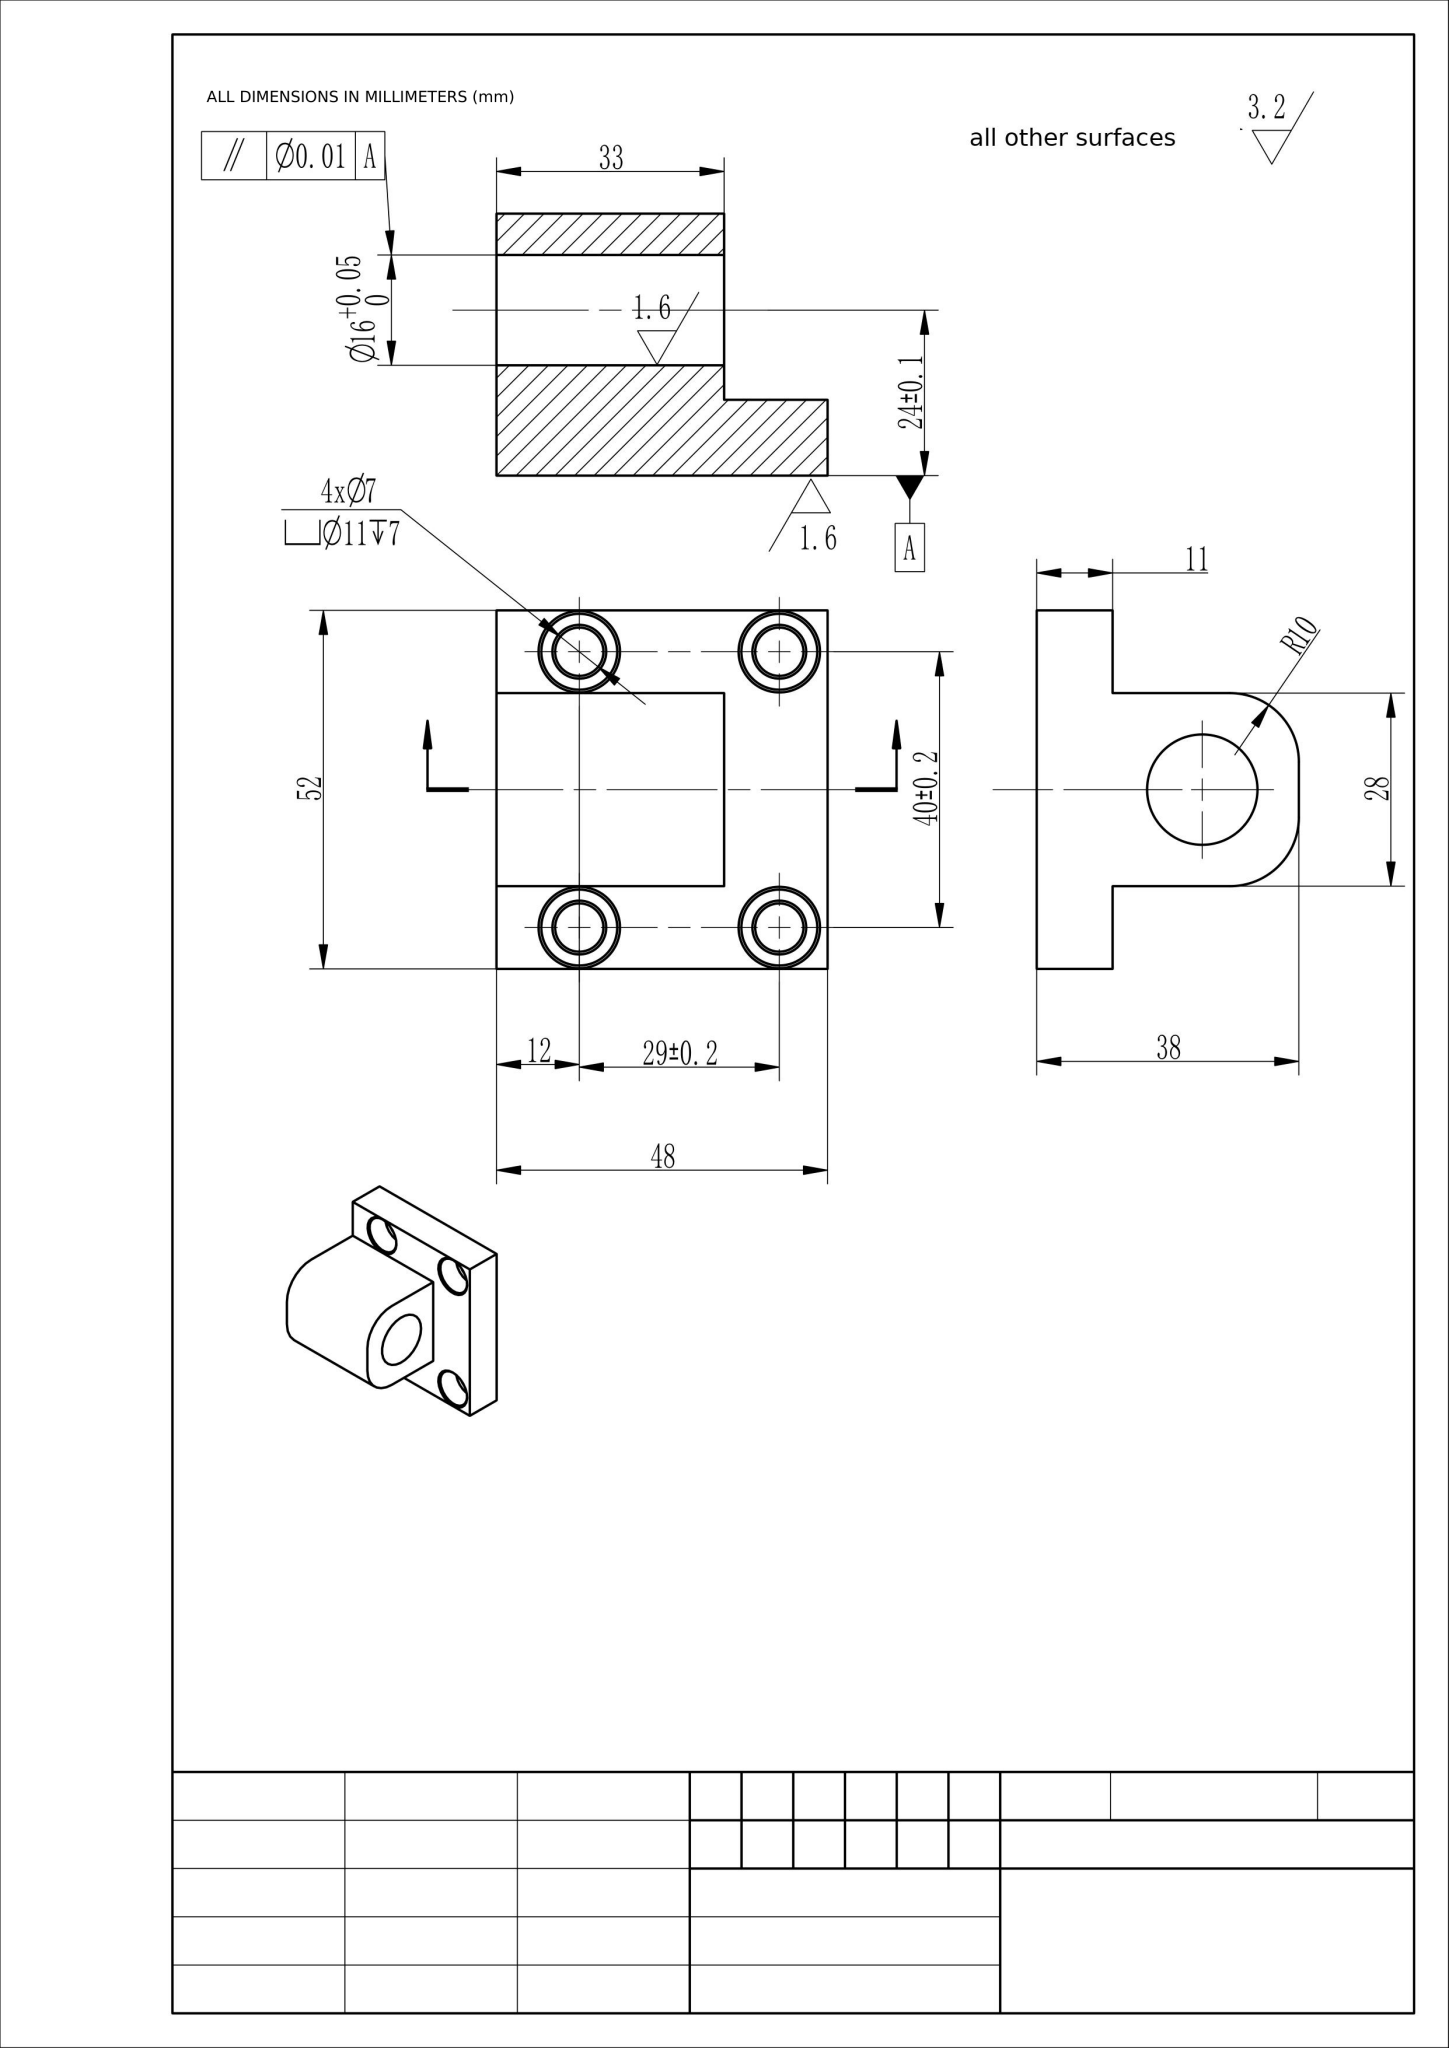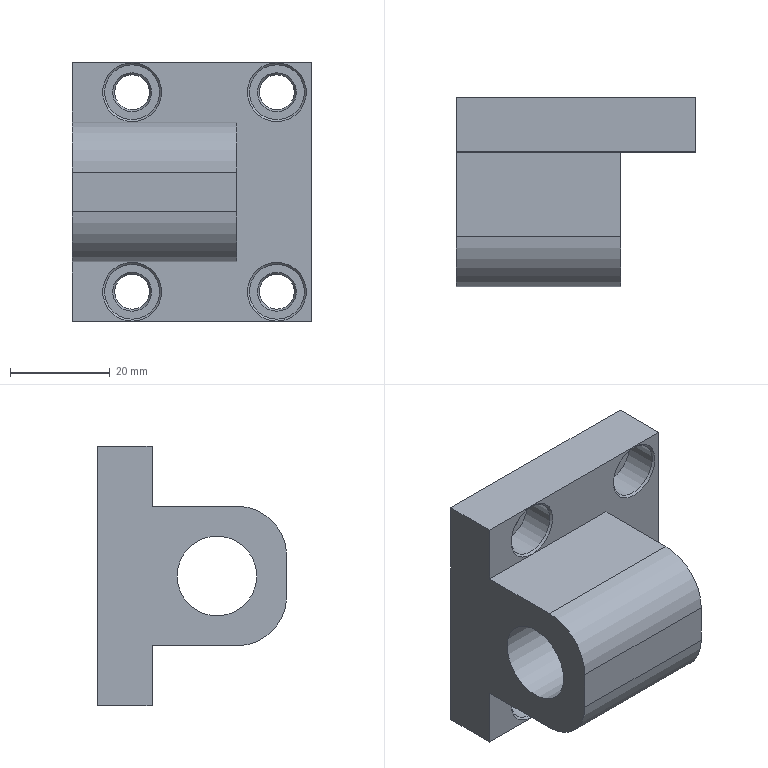Part | NX | mm | 1 solid | 37 faces | box 48 x 38 x 52 mm | volume 41090 mm3 | plane 14 | cone 12 | cylinder 11 | commonest cylinder face diameters 7 x4 11 x4 20 x2 16 x1
STEP:
#1=CARTESIAN_POINT('',(0.,0.,0.));
#2=DIRECTION('',(0.,0.,1.));
#3=DIRECTION('',(1.,0.,0.));
#4=AXIS2_PLACEMENT_3D('',#1,#2,#3);
#5=(LENGTH_UNIT()NAMED_UNIT(*)SI_UNIT(.MILLI.,.METRE.));
#6=UNCERTAINTY_MEASURE_WITH_UNIT(LENGTH_MEASURE(0.00002),#5,'','');
#7=(NAMED_UNIT(*)PLANE_ANGLE_UNIT()SI_UNIT($,.RADIAN.));
#8=PLANE_ANGLE_MEASURE_WITH_UNIT(PLANE_ANGLE_MEASURE(0.01745),#7);
#9=DIMENSIONAL_EXPONENTS(0.,0.,0.,0.,0.,0.,0.);
#10=(CONVERSION_BASED_UNIT('',#8)NAMED_UNIT(#9)PLANE_ANGLE_UNIT());
#11=(NAMED_UNIT(*)SI_UNIT($,.STERADIAN.)SOLID_ANGLE_UNIT());
#12=(GEOMETRIC_REPRESENTATION_CONTEXT(3)GLOBAL_UNCERTAINTY_ASSIGNED_CONTEXT((#6))GLOBAL_UNIT_ASSIGNED_CONTEXT((#5,#10,#11))REPRESENTATION_CONTEXT('',''));
#13=SHAPE_REPRESENTATION('',(#4),#12);
#14=CARTESIAN_POINT('',(0.,-14.,4.));
#15=VERTEX_POINT('',#14);
#16=CARTESIAN_POINT('',(0.,-14.,-4.));
#17=VERTEX_POINT('',#16);
#18=CARTESIAN_POINT('',(0.,-14.,14.));
#19=DIRECTION('',(0.,0.,-1.));
#20=VECTOR('',#19,1.);
#21=LINE('',#18,#20);
#22=EDGE_CURVE('',#15,#17,#21,.T.);
#23=ORIENTED_EDGE('',*,*,#22,.T.);
#24=CARTESIAN_POINT('',(33.,-14.,-4.));
#25=VERTEX_POINT('',#24);
#26=CARTESIAN_POINT('',(33.,-14.,-4.));
#27=DIRECTION('',(1.,0.,0.));
#28=VECTOR('',#27,1.);
#29=LINE('',#26,#28);
#30=EDGE_CURVE('',#17,#25,#29,.T.);
#31=ORIENTED_EDGE('',*,*,#30,.T.);
#32=CARTESIAN_POINT('',(33.,-14.,4.));
#33=VERTEX_POINT('',#32);
#34=CARTESIAN_POINT('',(33.,-14.,14.));
#35=DIRECTION('',(0.,0.,-1.));
#36=VECTOR('',#35,1.);
#37=LINE('',#34,#36);
#38=EDGE_CURVE('',#33,#25,#37,.T.);
#39=ORIENTED_EDGE('',*,*,#38,.F.);
#40=CARTESIAN_POINT('',(33.,-14.,4.));
#41=DIRECTION('',(-1.,0.,0.));
#42=VECTOR('',#41,1.);
#43=LINE('',#40,#42);
#44=EDGE_CURVE('',#33,#15,#43,.T.);
#45=ORIENTED_EDGE('',*,*,#44,.T.);
#46=EDGE_LOOP('',(#23,#31,#39,#45));
#47=FACE_OUTER_BOUND('',#46,.T.);
#48=CARTESIAN_POINT('',(33.,-14.,14.));
#49=DIRECTION('',(0.,1.,0.));
#50=DIRECTION('',(0.,0.,1.));
#51=AXIS2_PLACEMENT_3D('',#48,#49,#50);
#52=PLANE('',#51);
#53=ADVANCED_FACE('',(#47),#52,.F.);
#54=CARTESIAN_POINT('',(33.,-4.,-14.));
#55=VERTEX_POINT('',#54);
#56=CARTESIAN_POINT('',(33.,13.,-14.));
#57=VERTEX_POINT('',#56);
#58=CARTESIAN_POINT('',(33.,-14.,-14.));
#59=DIRECTION('',(0.,1.,0.));
#60=VECTOR('',#59,1.);
#61=LINE('',#58,#60);
#62=EDGE_CURVE('',#55,#57,#61,.T.);
#63=ORIENTED_EDGE('',*,*,#62,.F.);
#64=CARTESIAN_POINT('',(0.,-4.,-14.));
#65=VERTEX_POINT('',#64);
#66=CARTESIAN_POINT('',(33.,-4.,-14.));
#67=DIRECTION('',(-1.,0.,0.));
#68=VECTOR('',#67,1.);
#69=LINE('',#66,#68);
#70=EDGE_CURVE('',#55,#65,#69,.T.);
#71=ORIENTED_EDGE('',*,*,#70,.T.);
#72=CARTESIAN_POINT('',(0.,13.,-14.));
#73=VERTEX_POINT('',#72);
#74=CARTESIAN_POINT('',(0.,-14.,-14.));
#75=DIRECTION('',(0.,1.,0.));
#76=VECTOR('',#75,1.);
#77=LINE('',#74,#76);
#78=EDGE_CURVE('',#65,#73,#77,.T.);
#79=ORIENTED_EDGE('',*,*,#78,.T.);
#80=CARTESIAN_POINT('',(33.,13.,-14.));
#81=DIRECTION('',(-1.,0.,0.));
#82=VECTOR('',#81,1.);
#83=LINE('',#80,#82);
#84=EDGE_CURVE('',#57,#73,#83,.T.);
#85=ORIENTED_EDGE('',*,*,#84,.F.);
#86=EDGE_LOOP('',(#63,#71,#79,#85));
#87=FACE_OUTER_BOUND('',#86,.T.);
#88=CARTESIAN_POINT('',(33.,-14.,-14.));
#89=DIRECTION('',(0.,0.,1.));
#90=DIRECTION('',(1.,0.,0.));
#91=AXIS2_PLACEMENT_3D('',#88,#89,#90);
#92=PLANE('',#91);
#93=ADVANCED_FACE('',(#87),#92,.F.);
#94=CARTESIAN_POINT('',(0.,13.,-26.));
#95=VERTEX_POINT('',#94);
#96=CARTESIAN_POINT('',(0.,24.,-26.));
#97=VERTEX_POINT('',#96);
#98=CARTESIAN_POINT('',(0.,13.,-26.));
#99=DIRECTION('',(0.,1.,-0.));
#100=VECTOR('',#99,1.);
#101=LINE('',#98,#100);
#102=EDGE_CURVE('',#95,#97,#101,.T.);
#103=ORIENTED_EDGE('',*,*,#102,.T.);
#104=CARTESIAN_POINT('',(48.,24.,-26.));
#105=VERTEX_POINT('',#104);
#106=CARTESIAN_POINT('',(33.,24.,-26.));
#107=DIRECTION('',(-1.,0.,0.));
#108=VECTOR('',#107,1.);
#109=LINE('',#106,#108);
#110=EDGE_CURVE('',#105,#97,#109,.T.);
#111=ORIENTED_EDGE('',*,*,#110,.F.);
#112=CARTESIAN_POINT('',(48.,13.,-26.));
#113=VERTEX_POINT('',#112);
#114=CARTESIAN_POINT('',(48.,13.,-26.));
#115=DIRECTION('',(0.,1.,0.));
#116=VECTOR('',#115,1.);
#117=LINE('',#114,#116);
#118=EDGE_CURVE('',#113,#105,#117,.T.);
#119=ORIENTED_EDGE('',*,*,#118,.F.);
#120=CARTESIAN_POINT('',(33.,13.,-26.));
#121=DIRECTION('',(-1.,0.,0.));
#122=VECTOR('',#121,1.);
#123=LINE('',#120,#122);
#124=EDGE_CURVE('',#113,#95,#123,.T.);
#125=ORIENTED_EDGE('',*,*,#124,.T.);
#126=EDGE_LOOP('',(#103,#111,#119,#125));
#127=FACE_OUTER_BOUND('',#126,.T.);
#128=CARTESIAN_POINT('',(33.,13.,-26.));
#129=DIRECTION('',(0.,0.,1.));
#130=DIRECTION('',(0.,-1.,0.));
#131=AXIS2_PLACEMENT_3D('',#128,#129,#130);
#132=PLANE('',#131);
#133=ADVANCED_FACE('',(#127),#132,.F.);
#134=CARTESIAN_POINT('',(41.,24.,16.1));
#135=VERTEX_POINT('',#134);
#136=CARTESIAN_POINT('',(41.,24.,20.));
#137=DIRECTION('',(0.,-1.,0.));
#138=DIRECTION('',(0.,0.,-1.));
#139=AXIS2_PLACEMENT_3D('',#136,#137,#138);
#140=CIRCLE('',#139,3.9);
#141=EDGE_CURVE('',#135,#135,#140,.T.);
#142=ORIENTED_EDGE('',*,*,#141,.T.);
#143=EDGE_LOOP('',(#142));
#144=FACE_BOUND('',#143,.T.);
#145=CARTESIAN_POINT('',(41.,24.,-23.9));
#146=VERTEX_POINT('',#145);
#147=CARTESIAN_POINT('',(41.,24.,-20.));
#148=DIRECTION('',(0.,-1.,0.));
#149=DIRECTION('',(0.,0.,-1.));
#150=AXIS2_PLACEMENT_3D('',#147,#148,#149);
#151=CIRCLE('',#150,3.9);
#152=EDGE_CURVE('',#146,#146,#151,.T.);
#153=ORIENTED_EDGE('',*,*,#152,.T.);
#154=EDGE_LOOP('',(#153));
#155=FACE_BOUND('',#154,.T.);
#156=CARTESIAN_POINT('',(12.,24.,16.1));
#157=VERTEX_POINT('',#156);
#158=CARTESIAN_POINT('',(12.,24.,20.));
#159=DIRECTION('',(0.,-1.,0.));
#160=DIRECTION('',(0.,0.,-1.));
#161=AXIS2_PLACEMENT_3D('',#158,#159,#160);
#162=CIRCLE('',#161,3.9);
#163=EDGE_CURVE('',#157,#157,#162,.T.);
#164=ORIENTED_EDGE('',*,*,#163,.T.);
#165=EDGE_LOOP('',(#164));
#166=FACE_BOUND('',#165,.T.);
#167=CARTESIAN_POINT('',(12.,24.,-23.9));
#168=VERTEX_POINT('',#167);
#169=CARTESIAN_POINT('',(12.,24.,-20.));
#170=DIRECTION('',(0.,-1.,0.));
#171=DIRECTION('',(0.,0.,-1.));
#172=AXIS2_PLACEMENT_3D('',#169,#170,#171);
#173=CIRCLE('',#172,3.9);
#174=EDGE_CURVE('',#168,#168,#173,.T.);
#175=ORIENTED_EDGE('',*,*,#174,.T.);
#176=EDGE_LOOP('',(#175));
#177=FACE_BOUND('',#176,.T.);
#178=CARTESIAN_POINT('',(0.,24.,26.));
#179=VERTEX_POINT('',#178);
#180=CARTESIAN_POINT('',(0.,24.,-26.));
#181=DIRECTION('',(0.,0.,1.));
#182=VECTOR('',#181,1.);
#183=LINE('',#180,#182);
#184=EDGE_CURVE('',#97,#179,#183,.T.);
#185=ORIENTED_EDGE('',*,*,#184,.T.);
#186=CARTESIAN_POINT('',(48.,24.,26.));
#187=VERTEX_POINT('',#186);
#188=CARTESIAN_POINT('',(33.,24.,26.));
#189=DIRECTION('',(-1.,0.,0.));
#190=VECTOR('',#189,1.);
#191=LINE('',#188,#190);
#192=EDGE_CURVE('',#187,#179,#191,.T.);
#193=ORIENTED_EDGE('',*,*,#192,.F.);
#194=CARTESIAN_POINT('',(48.,24.,-26.));
#195=DIRECTION('',(0.,0.,1.));
#196=VECTOR('',#195,1.);
#197=LINE('',#194,#196);
#198=EDGE_CURVE('',#105,#187,#197,.T.);
#199=ORIENTED_EDGE('',*,*,#198,.F.);
#200=ORIENTED_EDGE('',*,*,#110,.T.);
#201=EDGE_LOOP('',(#185,#193,#199,#200));
#202=FACE_BOUND('',#201,.T.);
#203=CARTESIAN_POINT('',(33.,24.,-26.));
#204=DIRECTION('',(0.,-1.,0.));
#205=DIRECTION('',(0.,0.,-1.));
#206=AXIS2_PLACEMENT_3D('',#203,#204,#205);
#207=PLANE('',#206);
#208=ADVANCED_FACE('',(#144,#155,#166,#177,#202),#207,.F.);
#209=CARTESIAN_POINT('',(0.,13.,26.));
#210=VERTEX_POINT('',#209);
#211=CARTESIAN_POINT('',(0.,24.,26.));
#212=DIRECTION('',(0.,-1.,0.));
#213=VECTOR('',#212,1.);
#214=LINE('',#211,#213);
#215=EDGE_CURVE('',#179,#210,#214,.T.);
#216=ORIENTED_EDGE('',*,*,#215,.T.);
#217=CARTESIAN_POINT('',(48.,13.,26.));
#218=VERTEX_POINT('',#217);
#219=CARTESIAN_POINT('',(33.,13.,26.));
#220=DIRECTION('',(-1.,0.,0.));
#221=VECTOR('',#220,1.);
#222=LINE('',#219,#221);
#223=EDGE_CURVE('',#218,#210,#222,.T.);
#224=ORIENTED_EDGE('',*,*,#223,.F.);
#225=CARTESIAN_POINT('',(48.,24.,26.));
#226=DIRECTION('',(0.,-1.,-0.));
#227=VECTOR('',#226,1.);
#228=LINE('',#225,#227);
#229=EDGE_CURVE('',#187,#218,#228,.T.);
#230=ORIENTED_EDGE('',*,*,#229,.F.);
#231=ORIENTED_EDGE('',*,*,#192,.T.);
#232=EDGE_LOOP('',(#216,#224,#230,#231));
#233=FACE_OUTER_BOUND('',#232,.T.);
#234=CARTESIAN_POINT('',(33.,24.,26.));
#235=DIRECTION('',(0.,0.,-1.));
#236=DIRECTION('',(-1.,0.,0.));
#237=AXIS2_PLACEMENT_3D('',#234,#235,#236);
#238=PLANE('',#237);
#239=ADVANCED_FACE('',(#233),#238,.F.);
#240=CARTESIAN_POINT('',(41.,13.,25.9));
#241=VERTEX_POINT('',#240);
#242=CARTESIAN_POINT('',(41.,13.,20.));
#243=DIRECTION('',(0.,1.,0.));
#244=DIRECTION('',(0.,0.,1.));
#245=AXIS2_PLACEMENT_3D('',#242,#243,#244);
#246=CIRCLE('',#245,5.9);
#247=EDGE_CURVE('',#241,#241,#246,.T.);
#248=ORIENTED_EDGE('',*,*,#247,.T.);
#249=EDGE_LOOP('',(#248));
#250=FACE_BOUND('',#249,.T.);
#251=CARTESIAN_POINT('',(41.,13.,-14.1));
#252=VERTEX_POINT('',#251);
#253=CARTESIAN_POINT('',(41.,13.,-20.));
#254=DIRECTION('',(0.,1.,0.));
#255=DIRECTION('',(0.,0.,1.));
#256=AXIS2_PLACEMENT_3D('',#253,#254,#255);
#257=CIRCLE('',#256,5.9);
#258=EDGE_CURVE('',#252,#252,#257,.T.);
#259=ORIENTED_EDGE('',*,*,#258,.T.);
#260=EDGE_LOOP('',(#259));
#261=FACE_BOUND('',#260,.T.);
#262=CARTESIAN_POINT('',(12.,13.,25.9));
#263=VERTEX_POINT('',#262);
#264=CARTESIAN_POINT('',(12.,13.,20.));
#265=DIRECTION('',(0.,1.,0.));
#266=DIRECTION('',(0.,0.,1.));
#267=AXIS2_PLACEMENT_3D('',#264,#265,#266);
#268=CIRCLE('',#267,5.9);
#269=EDGE_CURVE('',#263,#263,#268,.T.);
#270=ORIENTED_EDGE('',*,*,#269,.T.);
#271=EDGE_LOOP('',(#270));
#272=FACE_BOUND('',#271,.T.);
#273=CARTESIAN_POINT('',(12.,13.,-14.1));
#274=VERTEX_POINT('',#273);
#275=CARTESIAN_POINT('',(12.,13.,-20.));
#276=DIRECTION('',(0.,1.,0.));
#277=DIRECTION('',(0.,0.,1.));
#278=AXIS2_PLACEMENT_3D('',#275,#276,#277);
#279=CIRCLE('',#278,5.9);
#280=EDGE_CURVE('',#274,#274,#279,.T.);
#281=ORIENTED_EDGE('',*,*,#280,.T.);
#282=EDGE_LOOP('',(#281));
#283=FACE_BOUND('',#282,.T.);
#284=CARTESIAN_POINT('',(0.,13.,14.));
#285=VERTEX_POINT('',#284);
#286=CARTESIAN_POINT('',(0.,13.,26.));
#287=DIRECTION('',(0.,0.,-1.));
#288=VECTOR('',#287,1.);
#289=LINE('',#286,#288);
#290=EDGE_CURVE('',#210,#285,#289,.T.);
#291=ORIENTED_EDGE('',*,*,#290,.T.);
#292=CARTESIAN_POINT('',(33.,13.,14.));
#293=VERTEX_POINT('',#292);
#294=CARTESIAN_POINT('',(33.,13.,14.));
#295=DIRECTION('',(-1.,0.,0.));
#296=VECTOR('',#295,1.);
#297=LINE('',#294,#296);
#298=EDGE_CURVE('',#293,#285,#297,.T.);
#299=ORIENTED_EDGE('',*,*,#298,.F.);
#300=CARTESIAN_POINT('',(33.,13.,26.));
#301=DIRECTION('',(0.,0.,1.));
#302=VECTOR('',#301,1.);
#303=LINE('',#300,#302);
#304=EDGE_CURVE('',#57,#293,#303,.T.);
#305=ORIENTED_EDGE('',*,*,#304,.F.);
#306=ORIENTED_EDGE('',*,*,#84,.T.);
#307=CARTESIAN_POINT('',(0.,13.,-14.));
#308=DIRECTION('',(0.,0.,-1.));
#309=VECTOR('',#308,1.);
#310=LINE('',#307,#309);
#311=EDGE_CURVE('',#73,#95,#310,.T.);
#312=ORIENTED_EDGE('',*,*,#311,.T.);
#313=ORIENTED_EDGE('',*,*,#124,.F.);
#314=CARTESIAN_POINT('',(48.,13.,26.));
#315=DIRECTION('',(0.,-0.,-1.));
#316=VECTOR('',#315,1.);
#317=LINE('',#314,#316);
#318=EDGE_CURVE('',#218,#113,#317,.T.);
#319=ORIENTED_EDGE('',*,*,#318,.F.);
#320=ORIENTED_EDGE('',*,*,#223,.T.);
#321=EDGE_LOOP('',(#291,#299,#305,#306,#312,#313,#319,#320));
#322=FACE_BOUND('',#321,.T.);
#323=CARTESIAN_POINT('',(33.,13.,26.));
#324=DIRECTION('',(0.,1.,0.));
#325=DIRECTION('',(0.,0.,1.));
#326=AXIS2_PLACEMENT_3D('',#323,#324,#325);
#327=PLANE('',#326);
#328=ADVANCED_FACE('',(#250,#261,#272,#283,#322),#327,.F.);
#329=CARTESIAN_POINT('',(0.,-4.,14.));
#330=VERTEX_POINT('',#329);
#331=CARTESIAN_POINT('',(0.,13.,14.));
#332=DIRECTION('',(0.,-1.,0.));
#333=VECTOR('',#332,1.);
#334=LINE('',#331,#333);
#335=EDGE_CURVE('',#285,#330,#334,.T.);
#336=ORIENTED_EDGE('',*,*,#335,.T.);
#337=CARTESIAN_POINT('',(33.,-4.,14.));
#338=VERTEX_POINT('',#337);
#339=CARTESIAN_POINT('',(33.,-4.,14.));
#340=DIRECTION('',(1.,0.,0.));
#341=VECTOR('',#340,1.);
#342=LINE('',#339,#341);
#343=EDGE_CURVE('',#330,#338,#342,.T.);
#344=ORIENTED_EDGE('',*,*,#343,.T.);
#345=CARTESIAN_POINT('',(33.,13.,14.));
#346=DIRECTION('',(0.,-1.,0.));
#347=VECTOR('',#346,1.);
#348=LINE('',#345,#347);
#349=EDGE_CURVE('',#293,#338,#348,.T.);
#350=ORIENTED_EDGE('',*,*,#349,.F.);
#351=ORIENTED_EDGE('',*,*,#298,.T.);
#352=EDGE_LOOP('',(#336,#344,#350,#351));
#353=FACE_OUTER_BOUND('',#352,.T.);
#354=CARTESIAN_POINT('',(33.,13.,14.));
#355=DIRECTION('',(0.,0.,-1.));
#356=DIRECTION('',(-1.,0.,0.));
#357=AXIS2_PLACEMENT_3D('',#354,#355,#356);
#358=PLANE('',#357);
#359=ADVANCED_FACE('',(#353),#358,.F.);
#360=CARTESIAN_POINT('',(33.,8.,-0.));
#361=VERTEX_POINT('',#360);
#362=CARTESIAN_POINT('',(33.,0.,0.));
#363=DIRECTION('',(1.,0.,0.));
#364=DIRECTION('',(0.,1.,-0.));
#365=AXIS2_PLACEMENT_3D('',#362,#363,#364);
#366=CIRCLE('',#365,8.);
#367=EDGE_CURVE('',#361,#361,#366,.T.);
#368=ORIENTED_EDGE('',*,*,#367,.T.);
#369=EDGE_LOOP('',(#368));
#370=FACE_BOUND('',#369,.T.);
#371=CARTESIAN_POINT('',(0.,8.,-0.));
#372=VERTEX_POINT('',#371);
#373=CARTESIAN_POINT('',(0.,0.,0.));
#374=DIRECTION('',(1.,0.,0.));
#375=DIRECTION('',(0.,1.,-0.));
#376=AXIS2_PLACEMENT_3D('',#373,#374,#375);
#377=CIRCLE('',#376,8.);
#378=EDGE_CURVE('',#372,#372,#377,.T.);
#379=ORIENTED_EDGE('',*,*,#378,.F.);
#380=EDGE_LOOP('',(#379));
#381=FACE_BOUND('',#380,.T.);
#382=CARTESIAN_POINT('',(33.,0.,0.));
#383=DIRECTION('',(-1.,0.,0.));
#384=DIRECTION('',(0.,0.,1.));
#385=AXIS2_PLACEMENT_3D('',#382,#383,#384);
#386=CYLINDRICAL_SURFACE('',#385,8.);
#387=ADVANCED_FACE('',(#370,#381),#386,.F.);
#388=ORIENTED_EDGE('',*,*,#304,.T.);
#389=ORIENTED_EDGE('',*,*,#349,.T.);
#390=CARTESIAN_POINT('',(33.,-4.,4.));
#391=DIRECTION('',(1.,0.,0.));
#392=DIRECTION('',(0.,0.,-1.));
#393=AXIS2_PLACEMENT_3D('',#390,#391,#392);
#394=CIRCLE('',#393,10.);
#395=EDGE_CURVE('',#338,#33,#394,.T.);
#396=ORIENTED_EDGE('',*,*,#395,.T.);
#397=ORIENTED_EDGE('',*,*,#38,.T.);
#398=CARTESIAN_POINT('',(33.,-4.,-4.));
#399=DIRECTION('',(1.,0.,0.));
#400=DIRECTION('',(0.,0.,-1.));
#401=AXIS2_PLACEMENT_3D('',#398,#399,#400);
#402=CIRCLE('',#401,10.);
#403=EDGE_CURVE('',#25,#55,#402,.T.);
#404=ORIENTED_EDGE('',*,*,#403,.T.);
#405=ORIENTED_EDGE('',*,*,#62,.T.);
#406=EDGE_LOOP('',(#388,#389,#396,#397,#404,#405));
#407=FACE_BOUND('',#406,.T.);
#408=ORIENTED_EDGE('',*,*,#367,.F.);
#409=EDGE_LOOP('',(#408));
#410=FACE_BOUND('',#409,.T.);
#411=CARTESIAN_POINT('',(33.,0.,0.));
#412=DIRECTION('',(1.,0.,0.));
#413=DIRECTION('',(0.,0.,-1.));
#414=AXIS2_PLACEMENT_3D('',#411,#412,#413);
#415=PLANE('',#414);
#416=ADVANCED_FACE('',(#407,#410),#415,.T.);
#417=ORIENTED_EDGE('',*,*,#78,.F.);
#418=CARTESIAN_POINT('',(0.,-4.,-4.));
#419=DIRECTION('',(-1.,0.,0.));
#420=DIRECTION('',(0.,0.,-1.));
#421=AXIS2_PLACEMENT_3D('',#418,#419,#420);
#422=CIRCLE('',#421,10.);
#423=EDGE_CURVE('',#65,#17,#422,.T.);
#424=ORIENTED_EDGE('',*,*,#423,.T.);
#425=ORIENTED_EDGE('',*,*,#22,.F.);
#426=CARTESIAN_POINT('',(0.,-4.,4.));
#427=DIRECTION('',(-1.,0.,0.));
#428=DIRECTION('',(0.,0.,-1.));
#429=AXIS2_PLACEMENT_3D('',#426,#427,#428);
#430=CIRCLE('',#429,10.);
#431=EDGE_CURVE('',#15,#330,#430,.T.);
#432=ORIENTED_EDGE('',*,*,#431,.T.);
#433=ORIENTED_EDGE('',*,*,#335,.F.);
#434=ORIENTED_EDGE('',*,*,#290,.F.);
#435=ORIENTED_EDGE('',*,*,#215,.F.);
#436=ORIENTED_EDGE('',*,*,#184,.F.);
#437=ORIENTED_EDGE('',*,*,#102,.F.);
#438=ORIENTED_EDGE('',*,*,#311,.F.);
#439=EDGE_LOOP('',(#417,#424,#425,#432,#433,#434,#435,#436,#437,#438));
#440=FACE_BOUND('',#439,.T.);
#441=ORIENTED_EDGE('',*,*,#378,.T.);
#442=EDGE_LOOP('',(#441));
#443=FACE_BOUND('',#442,.T.);
#444=CARTESIAN_POINT('',(0.,0.,0.));
#445=DIRECTION('',(1.,0.,0.));
#446=DIRECTION('',(0.,0.,-1.));
#447=AXIS2_PLACEMENT_3D('',#444,#445,#446);
#448=PLANE('',#447);
#449=ADVANCED_FACE('',(#440,#443),#448,.F.);
#450=ORIENTED_EDGE('',*,*,#403,.F.);
#451=ORIENTED_EDGE('',*,*,#30,.F.);
#452=ORIENTED_EDGE('',*,*,#423,.F.);
#453=ORIENTED_EDGE('',*,*,#70,.F.);
#454=EDGE_LOOP('',(#450,#451,#452,#453));
#455=FACE_OUTER_BOUND('',#454,.T.);
#456=CARTESIAN_POINT('',(33.,-4.,-4.));
#457=DIRECTION('',(-1.,0.,0.));
#458=DIRECTION('',(0.,0.,1.));
#459=AXIS2_PLACEMENT_3D('',#456,#457,#458);
#460=CYLINDRICAL_SURFACE('',#459,10.);
#461=ADVANCED_FACE('',(#455),#460,.T.);
#462=ORIENTED_EDGE('',*,*,#395,.F.);
#463=ORIENTED_EDGE('',*,*,#343,.F.);
#464=ORIENTED_EDGE('',*,*,#431,.F.);
#465=ORIENTED_EDGE('',*,*,#44,.F.);
#466=EDGE_LOOP('',(#462,#463,#464,#465));
#467=FACE_OUTER_BOUND('',#466,.T.);
#468=CARTESIAN_POINT('',(33.,-4.,4.));
#469=DIRECTION('',(-1.,0.,0.));
#470=DIRECTION('',(0.,0.,1.));
#471=AXIS2_PLACEMENT_3D('',#468,#469,#470);
#472=CYLINDRICAL_SURFACE('',#471,10.);
#473=ADVANCED_FACE('',(#467),#472,.T.);
#474=ORIENTED_EDGE('',*,*,#318,.T.);
#475=ORIENTED_EDGE('',*,*,#118,.T.);
#476=ORIENTED_EDGE('',*,*,#198,.T.);
#477=ORIENTED_EDGE('',*,*,#229,.T.);
#478=EDGE_LOOP('',(#474,#475,#476,#477));
#479=FACE_OUTER_BOUND('',#478,.T.);
#480=CARTESIAN_POINT('',(48.,0.,0.));
#481=DIRECTION('',(1.,0.,0.));
#482=DIRECTION('',(0.,0.,-1.));
#483=AXIS2_PLACEMENT_3D('',#480,#481,#482);
#484=PLANE('',#483);
#485=ADVANCED_FACE('',(#479),#484,.T.);
#486=CARTESIAN_POINT('',(12.,23.6,-23.5));
#487=VERTEX_POINT('',#486);
#488=CARTESIAN_POINT('',(12.,23.6,-20.));
#489=DIRECTION('',(0.,1.,0.));
#490=DIRECTION('',(0.,0.,-1.));
#491=AXIS2_PLACEMENT_3D('',#488,#489,#490);
#492=CIRCLE('',#491,3.5);
#493=EDGE_CURVE('',#487,#487,#492,.T.);
#494=ORIENTED_EDGE('',*,*,#493,.T.);
#495=EDGE_LOOP('',(#494));
#496=FACE_BOUND('',#495,.T.);
#497=CARTESIAN_POINT('',(12.,20.493,-16.5));
#498=VERTEX_POINT('',#497);
#499=CARTESIAN_POINT('',(12.,20.493,-20.));
#500=DIRECTION('',(0.,-1.,0.));
#501=DIRECTION('',(0.,0.,1.));
#502=AXIS2_PLACEMENT_3D('',#499,#500,#501);
#503=CIRCLE('',#502,3.5);
#504=EDGE_CURVE('',#498,#498,#503,.T.);
#505=ORIENTED_EDGE('',*,*,#504,.T.);
#506=EDGE_LOOP('',(#505));
#507=FACE_BOUND('',#506,.T.);
#508=CARTESIAN_POINT('',(12.,93.,-20.));
#509=DIRECTION('',(0.,1.,0.));
#510=DIRECTION('',(0.,0.,1.));
#511=AXIS2_PLACEMENT_3D('',#508,#509,#510);
#512=CYLINDRICAL_SURFACE('',#511,3.5);
#513=ADVANCED_FACE('',(#496,#507),#512,.F.);
#514=CARTESIAN_POINT('',(12.,19.8,-16.1));
#515=VERTEX_POINT('',#514);
#516=CARTESIAN_POINT('',(12.,19.8,-20.));
#517=DIRECTION('',(0.,1.,0.));
#518=DIRECTION('',(0.,0.,1.));
#519=AXIS2_PLACEMENT_3D('',#516,#517,#518);
#520=CIRCLE('',#519,3.9);
#521=EDGE_CURVE('',#515,#515,#520,.T.);
#522=ORIENTED_EDGE('',*,*,#521,.T.);
#523=EDGE_LOOP('',(#522));
#524=FACE_BOUND('',#523,.T.);
#525=CARTESIAN_POINT('',(12.,19.8,-14.5));
#526=VERTEX_POINT('',#525);
#527=CARTESIAN_POINT('',(12.,19.8,-20.));
#528=DIRECTION('',(0.,-1.,-0.));
#529=DIRECTION('',(0.,0.,1.));
#530=AXIS2_PLACEMENT_3D('',#527,#528,#529);
#531=CIRCLE('',#530,5.5);
#532=EDGE_CURVE('',#526,#526,#531,.T.);
#533=ORIENTED_EDGE('',*,*,#532,.T.);
#534=EDGE_LOOP('',(#533));
#535=FACE_BOUND('',#534,.T.);
#536=CARTESIAN_POINT('',(12.,19.8,-20.));
#537=DIRECTION('',(0.,1.,0.));
#538=DIRECTION('',(0.,-0.,1.));
#539=AXIS2_PLACEMENT_3D('',#536,#537,#538);
#540=PLANE('',#539);
#541=ADVANCED_FACE('',(#524,#535),#540,.F.);
#542=CARTESIAN_POINT('',(12.,13.4,-14.5));
#543=VERTEX_POINT('',#542);
#544=CARTESIAN_POINT('',(12.,13.4,-20.));
#545=DIRECTION('',(0.,-1.,0.));
#546=DIRECTION('',(0.,0.,1.));
#547=AXIS2_PLACEMENT_3D('',#544,#545,#546);
#548=CIRCLE('',#547,5.5);
#549=EDGE_CURVE('',#543,#543,#548,.T.);
#550=ORIENTED_EDGE('',*,*,#549,.T.);
#551=EDGE_LOOP('',(#550));
#552=FACE_BOUND('',#551,.T.);
#553=ORIENTED_EDGE('',*,*,#532,.F.);
#554=EDGE_LOOP('',(#553));
#555=FACE_BOUND('',#554,.T.);
#556=CARTESIAN_POINT('',(12.,13.,-20.));
#557=DIRECTION('',(0.,1.,0.));
#558=DIRECTION('',(0.,0.,1.));
#559=AXIS2_PLACEMENT_3D('',#556,#557,#558);
#560=CYLINDRICAL_SURFACE('',#559,5.5);
#561=ADVANCED_FACE('',(#552,#555),#560,.F.);
#562=ORIENTED_EDGE('',*,*,#521,.F.);
#563=EDGE_LOOP('',(#562));
#564=FACE_BOUND('',#563,.T.);
#565=ORIENTED_EDGE('',*,*,#504,.F.);
#566=EDGE_LOOP('',(#565));
#567=FACE_BOUND('',#566,.T.);
#568=CARTESIAN_POINT('',(12.,20.493,-20.));
#569=DIRECTION('',(0.,-1.,0.));
#570=DIRECTION('',(0.,0.,-1.));
#571=AXIS2_PLACEMENT_3D('',#568,#569,#570);
#572=CONICAL_SURFACE('',#571,3.5,30.);
#573=ADVANCED_FACE('',(#564,#567),#572,.F.);
#574=ORIENTED_EDGE('',*,*,#549,.F.);
#575=EDGE_LOOP('',(#574));
#576=FACE_BOUND('',#575,.T.);
#577=ORIENTED_EDGE('',*,*,#280,.F.);
#578=EDGE_LOOP('',(#577));
#579=FACE_BOUND('',#578,.T.);
#580=CARTESIAN_POINT('',(12.,13.,-20.));
#581=DIRECTION('',(0.,-1.,0.));
#582=DIRECTION('',(0.,0.,-1.));
#583=AXIS2_PLACEMENT_3D('',#580,#581,#582);
#584=CONICAL_SURFACE('',#583,5.9,45.);
#585=ADVANCED_FACE('',(#576,#579),#584,.F.);
#586=ORIENTED_EDGE('',*,*,#493,.F.);
#587=EDGE_LOOP('',(#586));
#588=FACE_BOUND('',#587,.T.);
#589=ORIENTED_EDGE('',*,*,#174,.F.);
#590=EDGE_LOOP('',(#589));
#591=FACE_BOUND('',#590,.T.);
#592=CARTESIAN_POINT('',(12.,24.,-20.));
#593=DIRECTION('',(0.,1.,0.));
#594=DIRECTION('',(0.,0.,1.));
#595=AXIS2_PLACEMENT_3D('',#592,#593,#594);
#596=CONICAL_SURFACE('',#595,3.9,45.);
#597=ADVANCED_FACE('',(#588,#591),#596,.F.);
#598=CARTESIAN_POINT('',(12.,23.6,16.5));
#599=VERTEX_POINT('',#598);
#600=CARTESIAN_POINT('',(12.,23.6,20.));
#601=DIRECTION('',(0.,1.,0.));
#602=DIRECTION('',(0.,0.,-1.));
#603=AXIS2_PLACEMENT_3D('',#600,#601,#602);
#604=CIRCLE('',#603,3.5);
#605=EDGE_CURVE('',#599,#599,#604,.T.);
#606=ORIENTED_EDGE('',*,*,#605,.T.);
#607=EDGE_LOOP('',(#606));
#608=FACE_BOUND('',#607,.T.);
#609=CARTESIAN_POINT('',(12.,20.493,23.5));
#610=VERTEX_POINT('',#609);
#611=CARTESIAN_POINT('',(12.,20.493,20.));
#612=DIRECTION('',(0.,-1.,0.));
#613=DIRECTION('',(0.,0.,1.));
#614=AXIS2_PLACEMENT_3D('',#611,#612,#613);
#615=CIRCLE('',#614,3.5);
#616=EDGE_CURVE('',#610,#610,#615,.T.);
#617=ORIENTED_EDGE('',*,*,#616,.T.);
#618=EDGE_LOOP('',(#617));
#619=FACE_BOUND('',#618,.T.);
#620=CARTESIAN_POINT('',(12.,93.,20.));
#621=DIRECTION('',(0.,1.,0.));
#622=DIRECTION('',(0.,0.,1.));
#623=AXIS2_PLACEMENT_3D('',#620,#621,#622);
#624=CYLINDRICAL_SURFACE('',#623,3.5);
#625=ADVANCED_FACE('',(#608,#619),#624,.F.);
#626=CARTESIAN_POINT('',(12.,19.8,23.9));
#627=VERTEX_POINT('',#626);
#628=CARTESIAN_POINT('',(12.,19.8,20.));
#629=DIRECTION('',(0.,1.,0.));
#630=DIRECTION('',(0.,0.,1.));
#631=AXIS2_PLACEMENT_3D('',#628,#629,#630);
#632=CIRCLE('',#631,3.9);
#633=EDGE_CURVE('',#627,#627,#632,.T.);
#634=ORIENTED_EDGE('',*,*,#633,.T.);
#635=EDGE_LOOP('',(#634));
#636=FACE_BOUND('',#635,.T.);
#637=CARTESIAN_POINT('',(12.,19.8,25.5));
#638=VERTEX_POINT('',#637);
#639=CARTESIAN_POINT('',(12.,19.8,20.));
#640=DIRECTION('',(0.,-1.,-0.));
#641=DIRECTION('',(0.,0.,1.));
#642=AXIS2_PLACEMENT_3D('',#639,#640,#641);
#643=CIRCLE('',#642,5.5);
#644=EDGE_CURVE('',#638,#638,#643,.T.);
#645=ORIENTED_EDGE('',*,*,#644,.T.);
#646=EDGE_LOOP('',(#645));
#647=FACE_BOUND('',#646,.T.);
#648=CARTESIAN_POINT('',(12.,19.8,20.));
#649=DIRECTION('',(0.,1.,0.));
#650=DIRECTION('',(0.,-0.,1.));
#651=AXIS2_PLACEMENT_3D('',#648,#649,#650);
#652=PLANE('',#651);
#653=ADVANCED_FACE('',(#636,#647),#652,.F.);
#654=CARTESIAN_POINT('',(12.,13.4,25.5));
#655=VERTEX_POINT('',#654);
#656=CARTESIAN_POINT('',(12.,13.4,20.));
#657=DIRECTION('',(0.,-1.,0.));
#658=DIRECTION('',(0.,0.,1.));
#659=AXIS2_PLACEMENT_3D('',#656,#657,#658);
#660=CIRCLE('',#659,5.5);
#661=EDGE_CURVE('',#655,#655,#660,.T.);
#662=ORIENTED_EDGE('',*,*,#661,.T.);
#663=EDGE_LOOP('',(#662));
#664=FACE_BOUND('',#663,.T.);
#665=ORIENTED_EDGE('',*,*,#644,.F.);
#666=EDGE_LOOP('',(#665));
#667=FACE_BOUND('',#666,.T.);
#668=CARTESIAN_POINT('',(12.,13.,20.));
#669=DIRECTION('',(0.,1.,0.));
#670=DIRECTION('',(0.,0.,1.));
#671=AXIS2_PLACEMENT_3D('',#668,#669,#670);
#672=CYLINDRICAL_SURFACE('',#671,5.5);
#673=ADVANCED_FACE('',(#664,#667),#672,.F.);
#674=ORIENTED_EDGE('',*,*,#633,.F.);
#675=EDGE_LOOP('',(#674));
#676=FACE_BOUND('',#675,.T.);
#677=ORIENTED_EDGE('',*,*,#616,.F.);
#678=EDGE_LOOP('',(#677));
#679=FACE_BOUND('',#678,.T.);
#680=CARTESIAN_POINT('',(12.,20.493,20.));
#681=DIRECTION('',(0.,-1.,0.));
#682=DIRECTION('',(0.,0.,-1.));
#683=AXIS2_PLACEMENT_3D('',#680,#681,#682);
#684=CONICAL_SURFACE('',#683,3.5,30.);
#685=ADVANCED_FACE('',(#676,#679),#684,.F.);
#686=ORIENTED_EDGE('',*,*,#661,.F.);
#687=EDGE_LOOP('',(#686));
#688=FACE_BOUND('',#687,.T.);
#689=ORIENTED_EDGE('',*,*,#269,.F.);
#690=EDGE_LOOP('',(#689));
#691=FACE_BOUND('',#690,.T.);
#692=CARTESIAN_POINT('',(12.,13.,20.));
#693=DIRECTION('',(0.,-1.,0.));
#694=DIRECTION('',(0.,0.,-1.));
#695=AXIS2_PLACEMENT_3D('',#692,#693,#694);
#696=CONICAL_SURFACE('',#695,5.9,45.);
#697=ADVANCED_FACE('',(#688,#691),#696,.F.);
#698=ORIENTED_EDGE('',*,*,#605,.F.);
#699=EDGE_LOOP('',(#698));
#700=FACE_BOUND('',#699,.T.);
#701=ORIENTED_EDGE('',*,*,#163,.F.);
#702=EDGE_LOOP('',(#701));
#703=FACE_BOUND('',#702,.T.);
#704=CARTESIAN_POINT('',(12.,24.,20.));
#705=DIRECTION('',(0.,1.,0.));
#706=DIRECTION('',(0.,0.,1.));
#707=AXIS2_PLACEMENT_3D('',#704,#705,#706);
#708=CONICAL_SURFACE('',#707,3.9,45.);
#709=ADVANCED_FACE('',(#700,#703),#708,.F.);
#710=CARTESIAN_POINT('',(41.,23.6,-23.5));
#711=VERTEX_POINT('',#710);
#712=CARTESIAN_POINT('',(41.,23.6,-20.));
#713=DIRECTION('',(0.,1.,0.));
#714=DIRECTION('',(0.,0.,-1.));
#715=AXIS2_PLACEMENT_3D('',#712,#713,#714);
#716=CIRCLE('',#715,3.5);
#717=EDGE_CURVE('',#711,#711,#716,.T.);
#718=ORIENTED_EDGE('',*,*,#717,.T.);
#719=EDGE_LOOP('',(#718));
#720=FACE_BOUND('',#719,.T.);
#721=CARTESIAN_POINT('',(41.,20.493,-16.5));
#722=VERTEX_POINT('',#721);
#723=CARTESIAN_POINT('',(41.,20.493,-20.));
#724=DIRECTION('',(0.,-1.,0.));
#725=DIRECTION('',(0.,0.,1.));
#726=AXIS2_PLACEMENT_3D('',#723,#724,#725);
#727=CIRCLE('',#726,3.5);
#728=EDGE_CURVE('',#722,#722,#727,.T.);
#729=ORIENTED_EDGE('',*,*,#728,.T.);
#730=EDGE_LOOP('',(#729));
#731=FACE_BOUND('',#730,.T.);
#732=CARTESIAN_POINT('',(41.,93.,-20.));
#733=DIRECTION('',(0.,1.,0.));
#734=DIRECTION('',(0.,0.,1.));
#735=AXIS2_PLACEMENT_3D('',#732,#733,#734);
#736=CYLINDRICAL_SURFACE('',#735,3.5);
#737=ADVANCED_FACE('',(#720,#731),#736,.F.);
#738=CARTESIAN_POINT('',(41.,19.8,-16.1));
#739=VERTEX_POINT('',#738);
#740=CARTESIAN_POINT('',(41.,19.8,-20.));
#741=DIRECTION('',(0.,1.,0.));
#742=DIRECTION('',(0.,0.,1.));
#743=AXIS2_PLACEMENT_3D('',#740,#741,#742);
#744=CIRCLE('',#743,3.9);
#745=EDGE_CURVE('',#739,#739,#744,.T.);
#746=ORIENTED_EDGE('',*,*,#745,.T.);
#747=EDGE_LOOP('',(#746));
#748=FACE_BOUND('',#747,.T.);
#749=CARTESIAN_POINT('',(41.,19.8,-14.5));
#750=VERTEX_POINT('',#749);
#751=CARTESIAN_POINT('',(41.,19.8,-20.));
#752=DIRECTION('',(0.,-1.,-0.));
#753=DIRECTION('',(0.,0.,1.));
#754=AXIS2_PLACEMENT_3D('',#751,#752,#753);
#755=CIRCLE('',#754,5.5);
#756=EDGE_CURVE('',#750,#750,#755,.T.);
#757=ORIENTED_EDGE('',*,*,#756,.T.);
#758=EDGE_LOOP('',(#757));
#759=FACE_BOUND('',#758,.T.);
#760=CARTESIAN_POINT('',(41.,19.8,-20.));
#761=DIRECTION('',(0.,1.,0.));
#762=DIRECTION('',(0.,-0.,1.));
#763=AXIS2_PLACEMENT_3D('',#760,#761,#762);
#764=PLANE('',#763);
#765=ADVANCED_FACE('',(#748,#759),#764,.F.);
#766=CARTESIAN_POINT('',(41.,13.4,-14.5));
#767=VERTEX_POINT('',#766);
#768=CARTESIAN_POINT('',(41.,13.4,-20.));
#769=DIRECTION('',(0.,-1.,0.));
#770=DIRECTION('',(0.,0.,1.));
#771=AXIS2_PLACEMENT_3D('',#768,#769,#770);
#772=CIRCLE('',#771,5.5);
#773=EDGE_CURVE('',#767,#767,#772,.T.);
#774=ORIENTED_EDGE('',*,*,#773,.T.);
#775=EDGE_LOOP('',(#774));
#776=FACE_BOUND('',#775,.T.);
#777=ORIENTED_EDGE('',*,*,#756,.F.);
#778=EDGE_LOOP('',(#777));
#779=FACE_BOUND('',#778,.T.);
#780=CARTESIAN_POINT('',(41.,13.,-20.));
#781=DIRECTION('',(0.,1.,0.));
#782=DIRECTION('',(0.,0.,1.));
#783=AXIS2_PLACEMENT_3D('',#780,#781,#782);
#784=CYLINDRICAL_SURFACE('',#783,5.5);
#785=ADVANCED_FACE('',(#776,#779),#784,.F.);
#786=ORIENTED_EDGE('',*,*,#745,.F.);
#787=EDGE_LOOP('',(#786));
#788=FACE_BOUND('',#787,.T.);
#789=ORIENTED_EDGE('',*,*,#728,.F.);
#790=EDGE_LOOP('',(#789));
#791=FACE_BOUND('',#790,.T.);
#792=CARTESIAN_POINT('',(41.,20.493,-20.));
#793=DIRECTION('',(0.,-1.,0.));
#794=DIRECTION('',(0.,0.,-1.));
#795=AXIS2_PLACEMENT_3D('',#792,#793,#794);
#796=CONICAL_SURFACE('',#795,3.5,30.);
#797=ADVANCED_FACE('',(#788,#791),#796,.F.);
#798=ORIENTED_EDGE('',*,*,#773,.F.);
#799=EDGE_LOOP('',(#798));
#800=FACE_BOUND('',#799,.T.);
#801=ORIENTED_EDGE('',*,*,#258,.F.);
#802=EDGE_LOOP('',(#801));
#803=FACE_BOUND('',#802,.T.);
#804=CARTESIAN_POINT('',(41.,13.,-20.));
#805=DIRECTION('',(0.,-1.,0.));
#806=DIRECTION('',(0.,0.,-1.));
#807=AXIS2_PLACEMENT_3D('',#804,#805,#806);
#808=CONICAL_SURFACE('',#807,5.9,45.);
#809=ADVANCED_FACE('',(#800,#803),#808,.F.);
#810=ORIENTED_EDGE('',*,*,#717,.F.);
#811=EDGE_LOOP('',(#810));
#812=FACE_BOUND('',#811,.T.);
#813=ORIENTED_EDGE('',*,*,#152,.F.);
#814=EDGE_LOOP('',(#813));
#815=FACE_BOUND('',#814,.T.);
#816=CARTESIAN_POINT('',(41.,24.,-20.));
#817=DIRECTION('',(0.,1.,0.));
#818=DIRECTION('',(0.,0.,1.));
#819=AXIS2_PLACEMENT_3D('',#816,#817,#818);
#820=CONICAL_SURFACE('',#819,3.9,45.);
#821=ADVANCED_FACE('',(#812,#815),#820,.F.);
#822=CARTESIAN_POINT('',(41.,23.6,16.5));
#823=VERTEX_POINT('',#822);
#824=CARTESIAN_POINT('',(41.,23.6,20.));
#825=DIRECTION('',(0.,1.,0.));
#826=DIRECTION('',(0.,0.,-1.));
#827=AXIS2_PLACEMENT_3D('',#824,#825,#826);
#828=CIRCLE('',#827,3.5);
#829=EDGE_CURVE('',#823,#823,#828,.T.);
#830=ORIENTED_EDGE('',*,*,#829,.T.);
#831=EDGE_LOOP('',(#830));
#832=FACE_BOUND('',#831,.T.);
#833=CARTESIAN_POINT('',(41.,20.493,23.5));
#834=VERTEX_POINT('',#833);
#835=CARTESIAN_POINT('',(41.,20.493,20.));
#836=DIRECTION('',(0.,-1.,0.));
#837=DIRECTION('',(0.,0.,1.));
#838=AXIS2_PLACEMENT_3D('',#835,#836,#837);
#839=CIRCLE('',#838,3.5);
#840=EDGE_CURVE('',#834,#834,#839,.T.);
#841=ORIENTED_EDGE('',*,*,#840,.T.);
#842=EDGE_LOOP('',(#841));
#843=FACE_BOUND('',#842,.T.);
#844=CARTESIAN_POINT('',(41.,93.,20.));
#845=DIRECTION('',(0.,1.,0.));
#846=DIRECTION('',(0.,0.,1.));
#847=AXIS2_PLACEMENT_3D('',#844,#845,#846);
#848=CYLINDRICAL_SURFACE('',#847,3.5);
#849=ADVANCED_FACE('',(#832,#843),#848,.F.);
#850=CARTESIAN_POINT('',(41.,19.8,23.9));
#851=VERTEX_POINT('',#850);
#852=CARTESIAN_POINT('',(41.,19.8,20.));
#853=DIRECTION('',(0.,1.,0.));
#854=DIRECTION('',(0.,0.,1.));
#855=AXIS2_PLACEMENT_3D('',#852,#853,#854);
#856=CIRCLE('',#855,3.9);
#857=EDGE_CURVE('',#851,#851,#856,.T.);
#858=ORIENTED_EDGE('',*,*,#857,.T.);
#859=EDGE_LOOP('',(#858));
#860=FACE_BOUND('',#859,.T.);
#861=CARTESIAN_POINT('',(41.,19.8,25.5));
#862=VERTEX_POINT('',#861);
#863=CARTESIAN_POINT('',(41.,19.8,20.));
#864=DIRECTION('',(0.,-1.,-0.));
#865=DIRECTION('',(0.,0.,1.));
#866=AXIS2_PLACEMENT_3D('',#863,#864,#865);
#867=CIRCLE('',#866,5.5);
#868=EDGE_CURVE('',#862,#862,#867,.T.);
#869=ORIENTED_EDGE('',*,*,#868,.T.);
#870=EDGE_LOOP('',(#869));
#871=FACE_BOUND('',#870,.T.);
#872=CARTESIAN_POINT('',(41.,19.8,20.));
#873=DIRECTION('',(0.,1.,0.));
#874=DIRECTION('',(0.,-0.,1.));
#875=AXIS2_PLACEMENT_3D('',#872,#873,#874);
#876=PLANE('',#875);
#877=ADVANCED_FACE('',(#860,#871),#876,.F.);
#878=CARTESIAN_POINT('',(41.,13.4,25.5));
#879=VERTEX_POINT('',#878);
#880=CARTESIAN_POINT('',(41.,13.4,20.));
#881=DIRECTION('',(0.,-1.,0.));
#882=DIRECTION('',(0.,0.,1.));
#883=AXIS2_PLACEMENT_3D('',#880,#881,#882);
#884=CIRCLE('',#883,5.5);
#885=EDGE_CURVE('',#879,#879,#884,.T.);
#886=ORIENTED_EDGE('',*,*,#885,.T.);
#887=EDGE_LOOP('',(#886));
#888=FACE_BOUND('',#887,.T.);
#889=ORIENTED_EDGE('',*,*,#868,.F.);
#890=EDGE_LOOP('',(#889));
#891=FACE_BOUND('',#890,.T.);
#892=CARTESIAN_POINT('',(41.,13.,20.));
#893=DIRECTION('',(0.,1.,0.));
#894=DIRECTION('',(0.,0.,1.));
#895=AXIS2_PLACEMENT_3D('',#892,#893,#894);
#896=CYLINDRICAL_SURFACE('',#895,5.5);
#897=ADVANCED_FACE('',(#888,#891),#896,.F.);
#898=ORIENTED_EDGE('',*,*,#857,.F.);
#899=EDGE_LOOP('',(#898));
#900=FACE_BOUND('',#899,.T.);
#901=ORIENTED_EDGE('',*,*,#840,.F.);
#902=EDGE_LOOP('',(#901));
#903=FACE_BOUND('',#902,.T.);
#904=CARTESIAN_POINT('',(41.,20.493,20.));
#905=DIRECTION('',(0.,-1.,0.));
#906=DIRECTION('',(0.,0.,-1.));
#907=AXIS2_PLACEMENT_3D('',#904,#905,#906);
#908=CONICAL_SURFACE('',#907,3.5,30.);
#909=ADVANCED_FACE('',(#900,#903),#908,.F.);
#910=ORIENTED_EDGE('',*,*,#885,.F.);
#911=EDGE_LOOP('',(#910));
#912=FACE_BOUND('',#911,.T.);
#913=ORIENTED_EDGE('',*,*,#247,.F.);
#914=EDGE_LOOP('',(#913));
#915=FACE_BOUND('',#914,.T.);
#916=CARTESIAN_POINT('',(41.,13.,20.));
#917=DIRECTION('',(0.,-1.,0.));
#918=DIRECTION('',(0.,0.,-1.));
#919=AXIS2_PLACEMENT_3D('',#916,#917,#918);
#920=CONICAL_SURFACE('',#919,5.9,45.);
#921=ADVANCED_FACE('',(#912,#915),#920,.F.);
#922=ORIENTED_EDGE('',*,*,#829,.F.);
#923=EDGE_LOOP('',(#922));
#924=FACE_BOUND('',#923,.T.);
#925=ORIENTED_EDGE('',*,*,#141,.F.);
#926=EDGE_LOOP('',(#925));
#927=FACE_BOUND('',#926,.T.);
#928=CARTESIAN_POINT('',(41.,24.,20.));
#929=DIRECTION('',(0.,1.,0.));
#930=DIRECTION('',(0.,0.,1.));
#931=AXIS2_PLACEMENT_3D('',#928,#929,#930);
#932=CONICAL_SURFACE('',#931,3.9,45.);
#933=ADVANCED_FACE('',(#924,#927),#932,.F.);
#934=CLOSED_SHELL('',(#53,#93,#133,#208,#239,#328,#359,#387,#416,#449,#461,#473,#485,#513,#541,#561,#573,#585,#597,#625,#653,#673,#685,#697,#709,#737,#765,#785,#797,#809,#821,#849,#877,#897,#909,#921,#933));
#935=MANIFOLD_SOLID_BREP('',#934);
#936=ADVANCED_BREP_SHAPE_REPRESENTATION('',(#935),#12);
#937=SHAPE_REPRESENTATION_RELATIONSHIP('','',#13,#936);
#938=PRESENTATION_LAYER_ASSIGNMENT('','',(#935));
#939=COLOUR_RGB('',1.,0.6,0.);
#940=FILL_AREA_STYLE_COLOUR('',#939);
#941=FILL_AREA_STYLE('',(#940));
#942=SURFACE_STYLE_FILL_AREA(#941);
#943=SURFACE_SIDE_STYLE('',(#942));
#944=SURFACE_STYLE_USAGE(.BOTH.,#943);
#945=PRESENTATION_STYLE_ASSIGNMENT((#944));
#946=STYLED_ITEM('',(#945),#935);
#947=MECHANICAL_DESIGN_GEOMETRIC_PRESENTATION_REPRESENTATION('',(#946),#12);